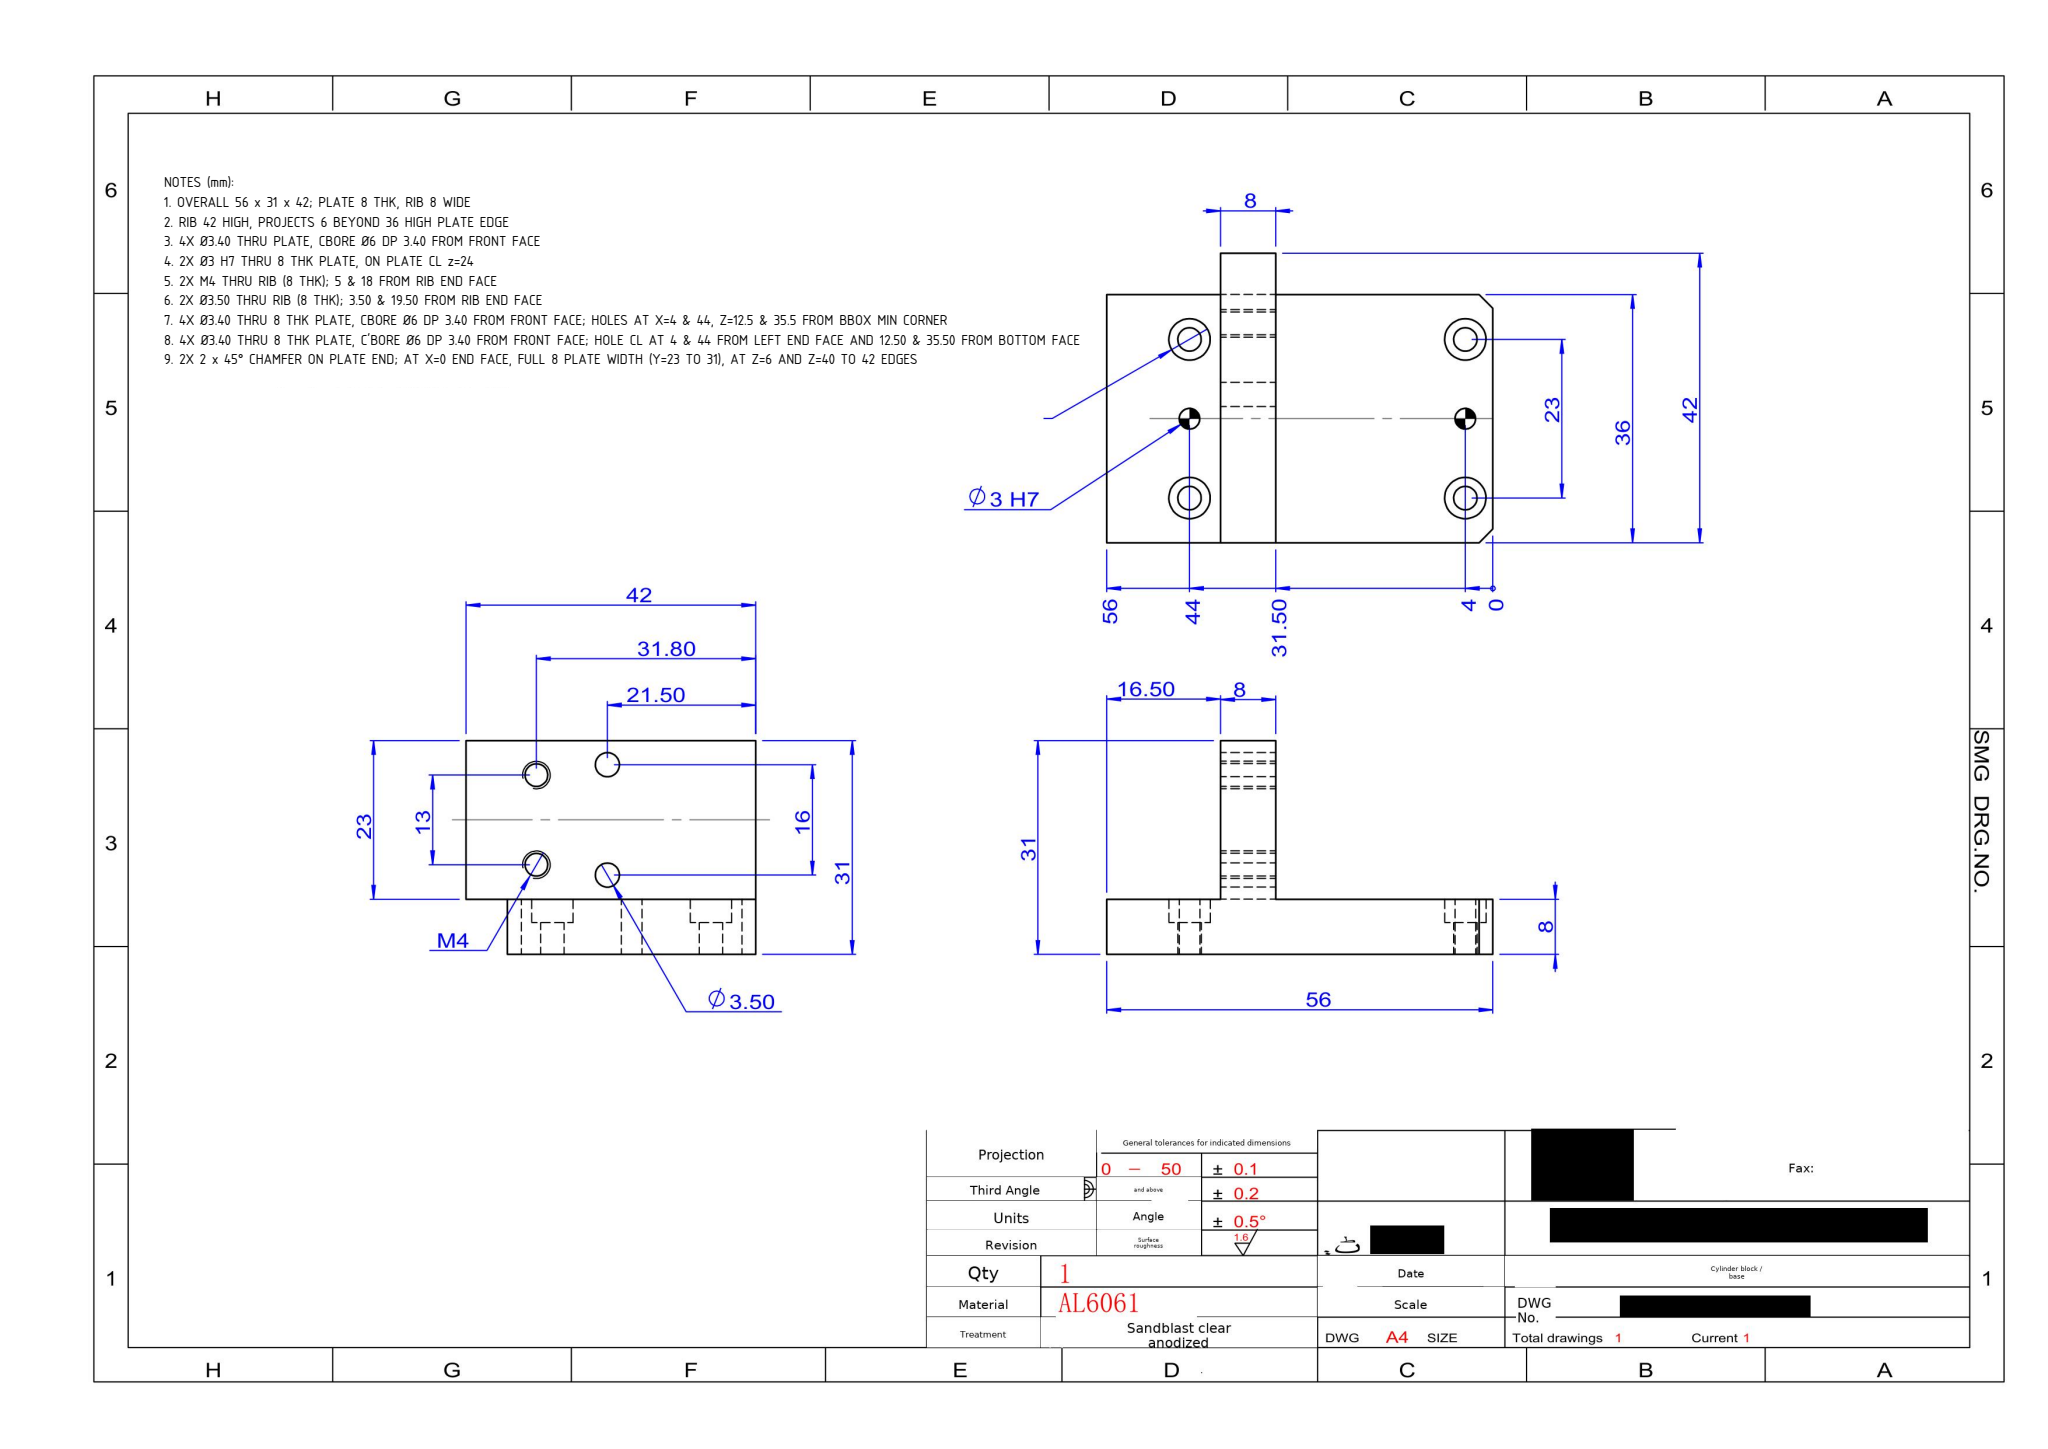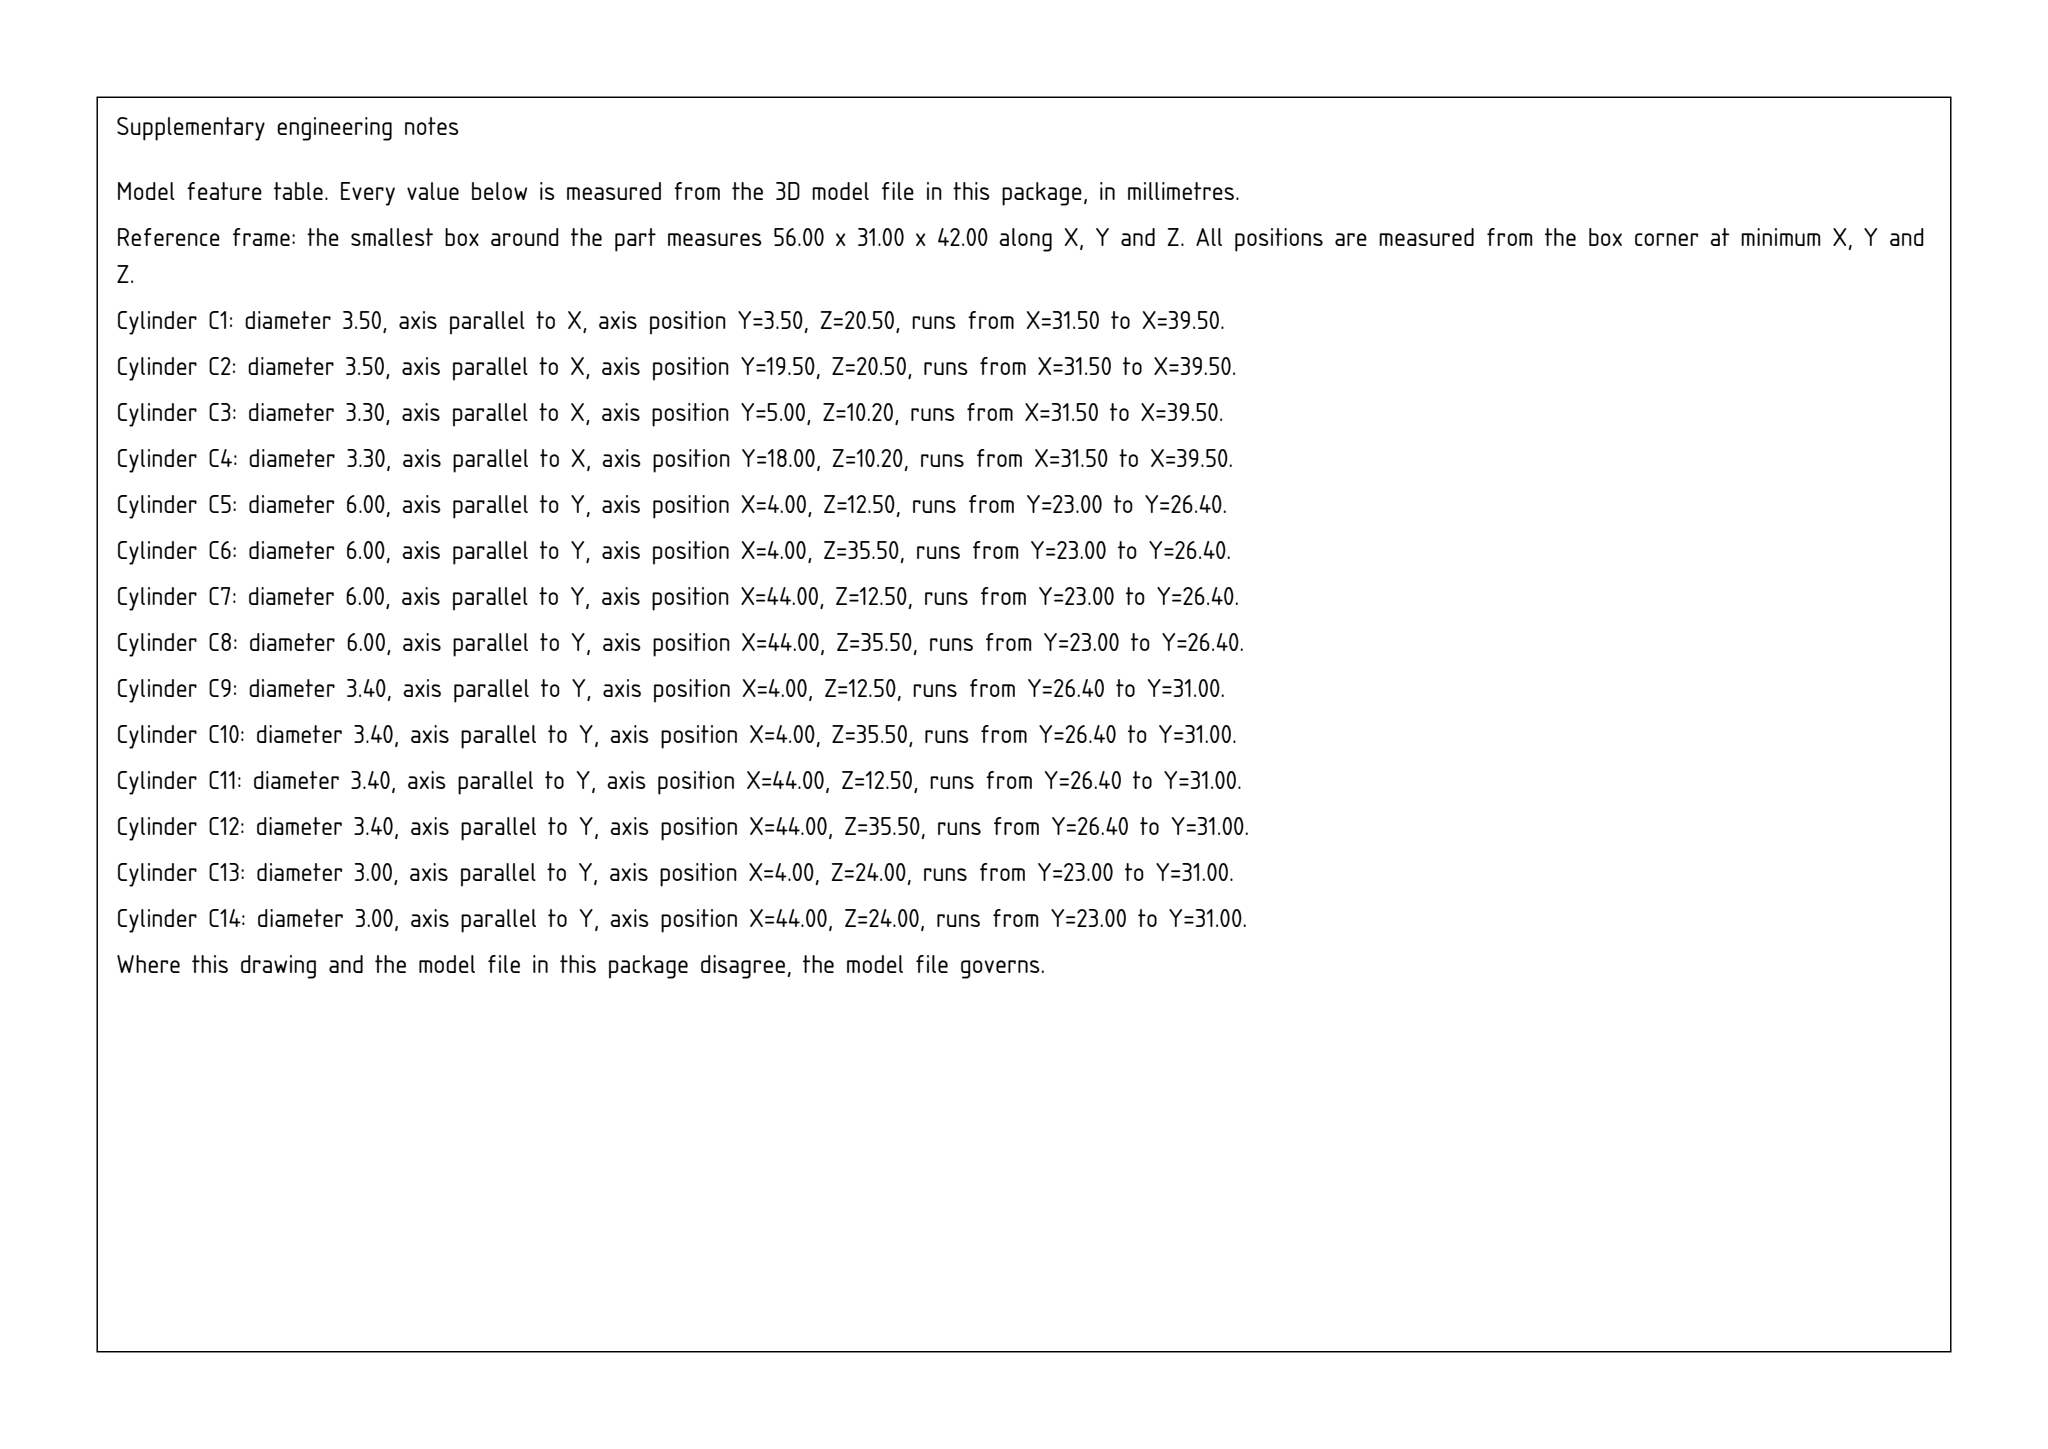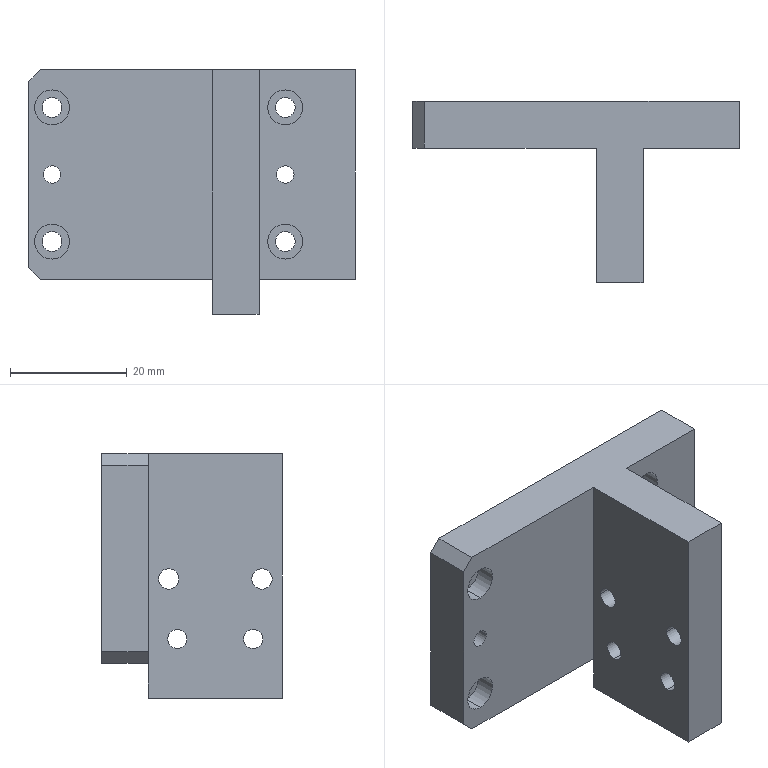Part | SolidWorks | mm | 1 solid | 46 faces | box 56 x 31 x 42 mm | volume 22869 mm3 | cylinder 28 | plane 18 | commonest cylinder face diameters 3.4 x8 6 x8 3 x4 3.5 x4 3.3 x4
Drawing notes:
OVERALL 56 x 31 x 42; PLATE 8 THK, RIB 8 WIDE | from the solid: bbox 56/31/42; y planes 23 & 31 (plate 8 thk); x planes 31.5 & 39.5 (rib 8 wide)
RIB 42 HIGH, PROJECTS 6 BEYOND 36 HIGH PLATE EDGE | from the solid: z planes 0, 6, 42: rib z0-42, plate z6-42 (36 high)
4X Ø3.40 THRU PLATE, CBORE Ø6 DP 3.40 FROM FRONT FACE | from the solid: Ø3.4 y-axis L4.6 + coaxial Ø6 y-axis L3.4 at x4/44, z12.5/35.5; 4.6+3.4=8 thk
2X Ø3 H7 THRU 8 THK PLATE, ON PLATE CL z=24 | from the solid: Ø3.0 y-axis cyls L8 at (x4,z24) and (x44,z24); plate y23-31
2X M4 THRU RIB (8 THK); 5 & 18 FROM RIB END FACE | from the solid: Ø3.3 tap drill x-axis cyls L8 at y5 & y18, z10.2, thru rib x31.5-39.5
2X Ø3.50 THRU RIB (8 THK); 3.50 & 19.50 FROM RIB END FACE | from the solid: Ø3.5 x-axis cyls L8 at y3.5 & y19.5, z20.5, thru rib x31.5-39.5
4X Ø3.40 THRU 8 THK PLATE, CBORE Ø6 DP 3.40 FROM FRONT FACE; HOLES AT X=4 & 44, Z=12.5 & 35.5 FROM BBOX MIN CORNER | from the solid: cylinders dia 3.4 axis y at (4,-,12.5),(4,-,35.5),(44,-,12.5),(44,-,35.5) len 4.6 and dia 6.0 axis y same positions len 3.4
4X Ø3.40 THRU 8 THK PLATE, C'BORE Ø6 DP 3.40 FROM FRONT FACE; HOLE CL AT 4 & 44 FROM LEFT END FACE AND 12.50 & 35.50 FROM BOTTOM FACE | from the solid: cylinders dia 3.40 axis y len 4.6 at (x=4,z=12.5),(4,35.5),(44,12.5),(44,35.5) with coaxial dia 6.0 axis y len 3.4 at same positions; plane y=26.4 (c'bore floor)
2X 2 x 45° CHAMFER ON PLATE END; AT X=0 END FACE, FULL 8 PLATE WIDTH (Y=23 TO 31), AT Z=6 AND Z=40 TO 42 EDGES | from the solid: inclined_planes: two 45.0/90.0/45.0 faces, bbox_from [0.0,23.0,40.0] and [0.0,23.0,6.0], size [2.0,8.0,2.0]